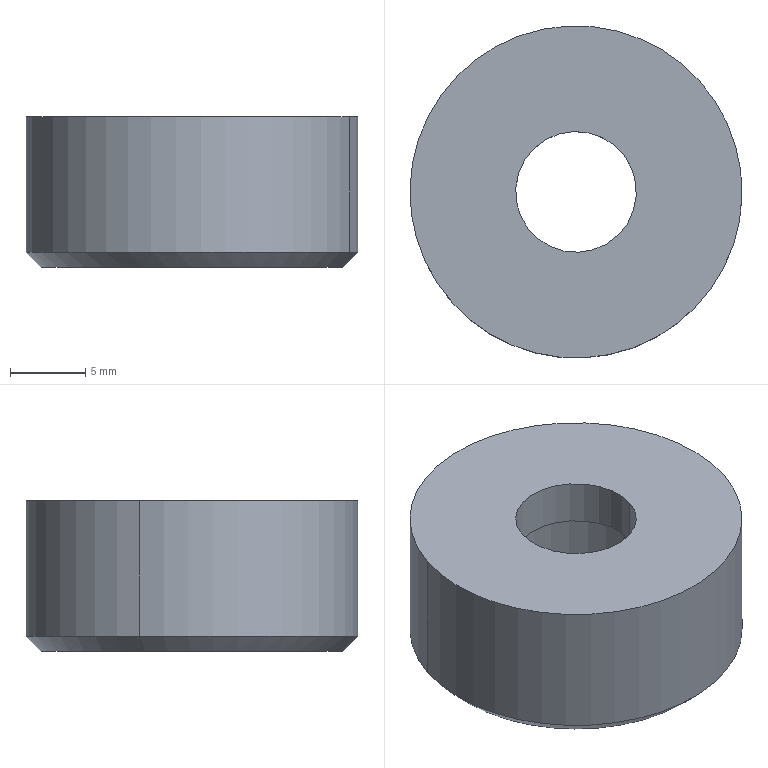Component | SolidWorks | DEM_R TEKER-1 | 1 solid | 11 faces | box 22 x 22 x 10 mm | volume 2758 mm3 | cylinder 6 | plane 3 | cone 2 | commonest cylinder face diameters 12.5 x2 22 x2 8 x2
build123d program:
from build123d import *

# Parameters (mm, degrees)
IZIM1_R                     = 11
Y_KSEKLIK_EKSTR_ZYON1_DEPTH = 10
IZIM2_R                     = 4
KES_EKSTR_ZYON1_DEPTH       = 10
IZIM3_R                     = 6.25
KES_EKSTR_ZYON2_DEPTH       = 7
CHAMFER1_SIZE               = 1


with BuildPart() as part:
    # izim1 → Y_kseklik-Ekstr_zyon1 (new body)
    with BuildSketch(Plane.XY):
        Circle(IZIM1_R)
    extrude(amount=Y_KSEKLIK_EKSTR_ZYON1_DEPTH)

    # izim2 → Kes-Ekstr_zyon1 (cut)
    with BuildSketch(Plane.XY.offset(10)):
        Circle(IZIM2_R)
    extrude(amount=-KES_EKSTR_ZYON1_DEPTH, mode=Mode.SUBTRACT)

    # izim3 → Kes-Ekstr_zyon2 (cut)
    with BuildSketch(Plane.XY.offset(10)):
        Circle(IZIM3_R)
    extrude(amount=-KES_EKSTR_ZYON2_DEPTH, mode=Mode.SUBTRACT)

    # Chamfer1
    chamfer1_edges = [part.edges().sort_by_distance(p)[0] for p in [
        (-11, 0, 10),
    ]]
    chamfer(chamfer1_edges, length=CHAMFER1_SIZE)


solid = part.part

# Placed as in the assembly
solid = solid.moved(Location((-146.473, 169.805, 183.974), (180, 0, 0)))
STEP:
#1=CARTESIAN_POINT('',(-5.393,6.561,6.849));
#2=VERTEX_POINT('',#1);
#3=CARTESIAN_POINT('',(-6.14,6.81,6.849));
#4=VERTEX_POINT('',#3);
#5=CARTESIAN_POINT('',(-5.767,6.685,6.849));
#6=DIRECTION('',(0.,-0.,-1.));
#7=DIRECTION('',(0.9488,-0.316,0.));
#8=AXIS2_PLACEMENT_3D('',#5,#6,#7);
#9=CIRCLE('',#8,0.3937);
#10=EDGE_CURVE('',#2,#4,#9,.T.);
#11=ORIENTED_EDGE('',*,*,#10,.F.);
#12=CARTESIAN_POINT('',(-5.356,6.548,6.889));
#13=VERTEX_POINT('',#12);
#14=CARTESIAN_POINT('',(-5.393,6.561,6.849));
#15=DIRECTION('',(0.6709,-0.2234,0.7071));
#16=VECTOR('',#15,39.37);
#17=LINE('',#14,#16);
#18=EDGE_CURVE('',#2,#13,#17,.T.);
#19=ORIENTED_EDGE('',*,*,#18,.T.);
#20=CARTESIAN_POINT('',(-6.178,6.822,6.889));
#21=VERTEX_POINT('',#20);
#22=CARTESIAN_POINT('',(-5.767,6.685,6.889));
#23=DIRECTION('',(-0.,0.,1.));
#24=DIRECTION('',(0.9488,-0.316,0.));
#25=AXIS2_PLACEMENT_3D('',#22,#23,#24);
#26=CIRCLE('',#25,0.4331);
#27=EDGE_CURVE('',#21,#13,#26,.T.);
#28=ORIENTED_EDGE('',*,*,#27,.F.);
#29=CARTESIAN_POINT('',(-6.14,6.81,6.849));
#30=DIRECTION('',(-0.6709,0.2234,0.7071));
#31=VECTOR('',#30,39.37);
#32=LINE('',#29,#31);
#33=EDGE_CURVE('',#4,#21,#32,.T.);
#34=ORIENTED_EDGE('',*,*,#33,.F.);
#35=EDGE_LOOP('',(#11,#19,#28,#34));
#36=FACE_OUTER_BOUND('',#35,.T.);
#37=CARTESIAN_POINT('',(-5.767,6.685,6.849));
#38=DIRECTION('',(-0.,0.,1.));
#39=DIRECTION('',(-0.9488,0.316,0.));
#40=AXIS2_PLACEMENT_3D('',#37,#38,#39);
#41=CONICAL_SURFACE('',#40,0.3937,0.7854);
#42=ADVANCED_FACE('',(#36),#41,.T.);
#43=CARTESIAN_POINT('',(-6.,6.763,7.125));
#44=VERTEX_POINT('',#43);
#45=CARTESIAN_POINT('',(-5.533,6.607,7.125));
#46=VERTEX_POINT('',#45);
#47=CARTESIAN_POINT('',(-5.767,6.685,7.125));
#48=DIRECTION('',(0.,-0.,-1.));
#49=DIRECTION('',(0.9488,-0.316,0.));
#50=AXIS2_PLACEMENT_3D('',#47,#48,#49);
#51=CIRCLE('',#50,0.2461);
#52=EDGE_CURVE('',#44,#46,#51,.T.);
#53=ORIENTED_EDGE('',*,*,#52,.F.);
#54=CARTESIAN_POINT('',(-6.,6.763,6.849));
#55=VERTEX_POINT('',#54);
#56=CARTESIAN_POINT('',(-6.,6.763,7.125));
#57=DIRECTION('',(0.,-0.,-1.));
#58=VECTOR('',#57,39.37);
#59=LINE('',#56,#58);
#60=EDGE_CURVE('',#44,#55,#59,.T.);
#61=ORIENTED_EDGE('',*,*,#60,.T.);
#62=CARTESIAN_POINT('',(-5.533,6.607,6.849));
#63=VERTEX_POINT('',#62);
#64=CARTESIAN_POINT('',(-5.767,6.685,6.849));
#65=DIRECTION('',(0.,-0.,-1.));
#66=DIRECTION('',(0.9488,-0.316,0.));
#67=AXIS2_PLACEMENT_3D('',#64,#65,#66);
#68=CIRCLE('',#67,0.2461);
#69=EDGE_CURVE('',#55,#63,#68,.T.);
#70=ORIENTED_EDGE('',*,*,#69,.T.);
#71=CARTESIAN_POINT('',(-5.533,6.607,7.125));
#72=DIRECTION('',(0.,-0.,-1.));
#73=VECTOR('',#72,39.37);
#74=LINE('',#71,#73);
#75=EDGE_CURVE('',#46,#63,#74,.T.);
#76=ORIENTED_EDGE('',*,*,#75,.F.);
#77=EDGE_LOOP('',(#53,#61,#70,#76));
#78=FACE_OUTER_BOUND('',#77,.T.);
#79=CARTESIAN_POINT('',(-5.767,6.685,7.125));
#80=DIRECTION('',(0.,-0.,-1.));
#81=DIRECTION('',(0.9488,-0.316,0.));
#82=AXIS2_PLACEMENT_3D('',#79,#80,#81);
#83=CYLINDRICAL_SURFACE('',#82,0.2461);
#84=ADVANCED_FACE('',(#78),#83,.F.);
#85=ORIENTED_EDGE('',*,*,#27,.T.);
#86=CARTESIAN_POINT('',(-5.356,6.548,7.243));
#87=VERTEX_POINT('',#86);
#88=CARTESIAN_POINT('',(-5.356,6.548,6.849));
#89=DIRECTION('',(-0.,0.,1.));
#90=VECTOR('',#89,39.37);
#91=LINE('',#88,#90);
#92=EDGE_CURVE('',#13,#87,#91,.T.);
#93=ORIENTED_EDGE('',*,*,#92,.T.);
#94=CARTESIAN_POINT('',(-6.178,6.822,7.243));
#95=VERTEX_POINT('',#94);
#96=CARTESIAN_POINT('',(-5.767,6.685,7.243));
#97=DIRECTION('',(0.,-0.,-1.));
#98=DIRECTION('',(0.9488,-0.316,0.));
#99=AXIS2_PLACEMENT_3D('',#96,#97,#98);
#100=CIRCLE('',#99,0.4331);
#101=EDGE_CURVE('',#87,#95,#100,.T.);
#102=ORIENTED_EDGE('',*,*,#101,.T.);
#103=CARTESIAN_POINT('',(-6.178,6.822,6.849));
#104=DIRECTION('',(-0.,0.,1.));
#105=VECTOR('',#104,39.37);
#106=LINE('',#103,#105);
#107=EDGE_CURVE('',#21,#95,#106,.T.);
#108=ORIENTED_EDGE('',*,*,#107,.F.);
#109=EDGE_LOOP('',(#85,#93,#102,#108));
#110=FACE_OUTER_BOUND('',#109,.T.);
#111=CARTESIAN_POINT('',(-5.767,6.685,6.849));
#112=DIRECTION('',(-0.,0.,1.));
#113=DIRECTION('',(-0.9488,0.316,0.));
#114=AXIS2_PLACEMENT_3D('',#111,#112,#113);
#115=CYLINDRICAL_SURFACE('',#114,0.4331);
#116=ADVANCED_FACE('',(#110),#115,.T.);
#117=CARTESIAN_POINT('',(-5.916,6.735,7.243));
#118=VERTEX_POINT('',#117);
#119=CARTESIAN_POINT('',(-5.617,6.635,7.243));
#120=VERTEX_POINT('',#119);
#121=CARTESIAN_POINT('',(-5.767,6.685,7.243));
#122=DIRECTION('',(0.,-0.,-1.));
#123=DIRECTION('',(0.9488,-0.316,0.));
#124=AXIS2_PLACEMENT_3D('',#121,#122,#123);
#125=CIRCLE('',#124,0.1575);
#126=EDGE_CURVE('',#118,#120,#125,.T.);
#127=ORIENTED_EDGE('',*,*,#126,.F.);
#128=CARTESIAN_POINT('',(-5.916,6.735,7.125));
#129=VERTEX_POINT('',#128);
#130=CARTESIAN_POINT('',(-5.916,6.735,7.243));
#131=DIRECTION('',(0.,-0.,-1.));
#132=VECTOR('',#131,39.37);
#133=LINE('',#130,#132);
#134=EDGE_CURVE('',#118,#129,#133,.T.);
#135=ORIENTED_EDGE('',*,*,#134,.T.);
#136=CARTESIAN_POINT('',(-5.617,6.635,7.125));
#137=VERTEX_POINT('',#136);
#138=CARTESIAN_POINT('',(-5.767,6.685,7.125));
#139=DIRECTION('',(-0.,0.,1.));
#140=DIRECTION('',(0.9488,-0.316,0.));
#141=AXIS2_PLACEMENT_3D('',#138,#139,#140);
#142=CIRCLE('',#141,0.1575);
#143=EDGE_CURVE('',#137,#129,#142,.T.);
#144=ORIENTED_EDGE('',*,*,#143,.F.);
#145=CARTESIAN_POINT('',(-5.617,6.635,7.243));
#146=DIRECTION('',(0.,-0.,-1.));
#147=VECTOR('',#146,39.37);
#148=LINE('',#145,#147);
#149=EDGE_CURVE('',#120,#137,#148,.T.);
#150=ORIENTED_EDGE('',*,*,#149,.F.);
#151=EDGE_LOOP('',(#127,#135,#144,#150));
#152=FACE_OUTER_BOUND('',#151,.T.);
#153=CARTESIAN_POINT('',(-5.767,6.685,7.243));
#154=DIRECTION('',(0.,-0.,-1.));
#155=DIRECTION('',(0.9488,-0.316,0.));
#156=AXIS2_PLACEMENT_3D('',#153,#154,#155);
#157=CYLINDRICAL_SURFACE('',#156,0.1575);
#158=ADVANCED_FACE('',(#152),#157,.F.);
#159=ORIENTED_EDGE('',*,*,#134,.F.);
#160=CARTESIAN_POINT('',(-5.767,6.685,7.243));
#161=DIRECTION('',(0.,-0.,-1.));
#162=DIRECTION('',(0.9488,-0.316,0.));
#163=AXIS2_PLACEMENT_3D('',#160,#161,#162);
#164=CIRCLE('',#163,0.1575);
#165=EDGE_CURVE('',#120,#118,#164,.T.);
#166=ORIENTED_EDGE('',*,*,#165,.F.);
#167=ORIENTED_EDGE('',*,*,#149,.T.);
#168=CARTESIAN_POINT('',(-5.767,6.685,7.125));
#169=DIRECTION('',(-0.,0.,1.));
#170=DIRECTION('',(0.9488,-0.316,0.));
#171=AXIS2_PLACEMENT_3D('',#168,#169,#170);
#172=CIRCLE('',#171,0.1575);
#173=EDGE_CURVE('',#129,#137,#172,.T.);
#174=ORIENTED_EDGE('',*,*,#173,.F.);
#175=EDGE_LOOP('',(#159,#166,#167,#174));
#176=FACE_OUTER_BOUND('',#175,.T.);
#177=CARTESIAN_POINT('',(-5.767,6.685,7.243));
#178=DIRECTION('',(0.,-0.,-1.));
#179=DIRECTION('',(0.9488,-0.316,0.));
#180=AXIS2_PLACEMENT_3D('',#177,#178,#179);
#181=CYLINDRICAL_SURFACE('',#180,0.1575);
#182=ADVANCED_FACE('',(#176),#181,.F.);
#183=ORIENTED_EDGE('',*,*,#92,.F.);
#184=CARTESIAN_POINT('',(-5.767,6.685,6.889));
#185=DIRECTION('',(-0.,0.,1.));
#186=DIRECTION('',(0.9488,-0.316,0.));
#187=AXIS2_PLACEMENT_3D('',#184,#185,#186);
#188=CIRCLE('',#187,0.4331);
#189=EDGE_CURVE('',#13,#21,#188,.T.);
#190=ORIENTED_EDGE('',*,*,#189,.T.);
#191=ORIENTED_EDGE('',*,*,#107,.T.);
#192=CARTESIAN_POINT('',(-5.767,6.685,7.243));
#193=DIRECTION('',(0.,-0.,-1.));
#194=DIRECTION('',(0.9488,-0.316,0.));
#195=AXIS2_PLACEMENT_3D('',#192,#193,#194);
#196=CIRCLE('',#195,0.4331);
#197=EDGE_CURVE('',#95,#87,#196,.T.);
#198=ORIENTED_EDGE('',*,*,#197,.T.);
#199=EDGE_LOOP('',(#183,#190,#191,#198));
#200=FACE_OUTER_BOUND('',#199,.T.);
#201=CARTESIAN_POINT('',(-5.767,6.685,6.849));
#202=DIRECTION('',(-0.,0.,1.));
#203=DIRECTION('',(-0.9488,0.316,0.));
#204=AXIS2_PLACEMENT_3D('',#201,#202,#203);
#205=CYLINDRICAL_SURFACE('',#204,0.4331);
#206=ADVANCED_FACE('',(#200),#205,.T.);
#207=CARTESIAN_POINT('',(-5.767,6.685,6.849));
#208=DIRECTION('',(0.,-0.,-1.));
#209=DIRECTION('',(0.9488,-0.316,0.));
#210=AXIS2_PLACEMENT_3D('',#207,#208,#209);
#211=CIRCLE('',#210,0.3937);
#212=EDGE_CURVE('',#4,#2,#211,.T.);
#213=ORIENTED_EDGE('',*,*,#212,.T.);
#214=ORIENTED_EDGE('',*,*,#10,.T.);
#215=EDGE_LOOP('',(#213,#214));
#216=FACE_OUTER_BOUND('',#215,.T.);
#217=CARTESIAN_POINT('',(-5.767,6.685,6.849));
#218=DIRECTION('',(0.,-0.,-1.));
#219=DIRECTION('',(0.9488,-0.316,0.));
#220=AXIS2_PLACEMENT_3D('',#217,#218,#219);
#221=CIRCLE('',#220,0.2461);
#222=EDGE_CURVE('',#63,#55,#221,.T.);
#223=ORIENTED_EDGE('',*,*,#222,.F.);
#224=ORIENTED_EDGE('',*,*,#69,.F.);
#225=EDGE_LOOP('',(#223,#224));
#226=FACE_BOUND('',#225,.T.);
#227=CARTESIAN_POINT('',(-5.767,6.685,6.849));
#228=DIRECTION('',(0.,-0.,-1.));
#229=DIRECTION('',(0.9488,-0.316,0.));
#230=AXIS2_PLACEMENT_3D('',#227,#228,#229);
#231=PLANE('',#230);
#232=ADVANCED_FACE('',(#216,#226),#231,.T.);
#233=ORIENTED_EDGE('',*,*,#165,.T.);
#234=ORIENTED_EDGE('',*,*,#126,.T.);
#235=EDGE_LOOP('',(#233,#234));
#236=FACE_BOUND('',#235,.T.);
#237=ORIENTED_EDGE('',*,*,#197,.F.);
#238=ORIENTED_EDGE('',*,*,#101,.F.);
#239=EDGE_LOOP('',(#237,#238));
#240=FACE_OUTER_BOUND('',#239,.T.);
#241=CARTESIAN_POINT('',(-5.767,6.685,7.243));
#242=DIRECTION('',(0.,-0.,-1.));
#243=DIRECTION('',(0.9488,-0.316,0.));
#244=AXIS2_PLACEMENT_3D('',#241,#242,#243);
#245=PLANE('',#244);
#246=ADVANCED_FACE('',(#236,#240),#245,.F.);
#247=CARTESIAN_POINT('',(-5.767,6.685,7.125));
#248=DIRECTION('',(0.,-0.,-1.));
#249=DIRECTION('',(0.9488,-0.316,0.));
#250=AXIS2_PLACEMENT_3D('',#247,#248,#249);
#251=CIRCLE('',#250,0.2461);
#252=EDGE_CURVE('',#46,#44,#251,.T.);
#253=ORIENTED_EDGE('',*,*,#252,.T.);
#254=ORIENTED_EDGE('',*,*,#52,.T.);
#255=EDGE_LOOP('',(#253,#254));
#256=FACE_OUTER_BOUND('',#255,.T.);
#257=ORIENTED_EDGE('',*,*,#143,.T.);
#258=ORIENTED_EDGE('',*,*,#173,.T.);
#259=EDGE_LOOP('',(#257,#258));
#260=FACE_BOUND('',#259,.T.);
#261=CARTESIAN_POINT('',(-5.767,6.685,7.125));
#262=DIRECTION('',(0.,-0.,-1.));
#263=DIRECTION('',(0.9488,-0.316,0.));
#264=AXIS2_PLACEMENT_3D('',#261,#262,#263);
#265=PLANE('',#264);
#266=ADVANCED_FACE('',(#256,#260),#265,.T.);
#267=ORIENTED_EDGE('',*,*,#60,.F.);
#268=ORIENTED_EDGE('',*,*,#252,.F.);
#269=ORIENTED_EDGE('',*,*,#75,.T.);
#270=ORIENTED_EDGE('',*,*,#222,.T.);
#271=EDGE_LOOP('',(#267,#268,#269,#270));
#272=FACE_OUTER_BOUND('',#271,.T.);
#273=CARTESIAN_POINT('',(-5.767,6.685,7.125));
#274=DIRECTION('',(0.,-0.,-1.));
#275=DIRECTION('',(0.9488,-0.316,0.));
#276=AXIS2_PLACEMENT_3D('',#273,#274,#275);
#277=CYLINDRICAL_SURFACE('',#276,0.2461);
#278=ADVANCED_FACE('',(#272),#277,.F.);
#279=ORIENTED_EDGE('',*,*,#18,.F.);
#280=ORIENTED_EDGE('',*,*,#212,.F.);
#281=ORIENTED_EDGE('',*,*,#33,.T.);
#282=ORIENTED_EDGE('',*,*,#189,.F.);
#283=EDGE_LOOP('',(#279,#280,#281,#282));
#284=FACE_OUTER_BOUND('',#283,.T.);
#285=CARTESIAN_POINT('',(-5.767,6.685,6.849));
#286=DIRECTION('',(-0.,0.,1.));
#287=DIRECTION('',(-0.9488,0.316,0.));
#288=AXIS2_PLACEMENT_3D('',#285,#286,#287);
#289=CONICAL_SURFACE('',#288,0.3937,0.7854);
#290=ADVANCED_FACE('',(#284),#289,.T.);
#291=CLOSED_SHELL('',(#42,#84,#116,#158,#182,#206,#232,#246,#266,#278,#290));
#292=MANIFOLD_SOLID_BREP('',#291);
#293=CARTESIAN_POINT('',(0.,0.,0.));
#294=DIRECTION('',(0.,0.,1.));
#295=DIRECTION('',(1.,0.,0.));
#296=AXIS2_PLACEMENT_3D('',#293,#294,#295);
#297=(LENGTH_UNIT()NAMED_UNIT(*)SI_UNIT($,.METRE.));
#298=LENGTH_MEASURE_WITH_UNIT(LENGTH_MEASURE(0.0254),#297);
#299=DIMENSIONAL_EXPONENTS(1.,0.,0.,0.,0.,0.,0.);
#300=(CONVERSION_BASED_UNIT('',#298)LENGTH_UNIT()NAMED_UNIT(#299));
#301=UNCERTAINTY_MEASURE_WITH_UNIT(LENGTH_MEASURE(0.00001),#300,'','');
#302=(NAMED_UNIT(*)PLANE_ANGLE_UNIT()SI_UNIT($,.RADIAN.));
#303=(NAMED_UNIT(*)SI_UNIT($,.STERADIAN.)SOLID_ANGLE_UNIT());
#304=(GEOMETRIC_REPRESENTATION_CONTEXT(3)GLOBAL_UNCERTAINTY_ASSIGNED_CONTEXT((#301))GLOBAL_UNIT_ASSIGNED_CONTEXT((#300,#302,#303))REPRESENTATION_CONTEXT('',''));
#305=ADVANCED_BREP_SHAPE_REPRESENTATION('',(#292,#296),#304);
#306=COLOUR_RGB('',0.7922,0.8196,0.9333);
#307=FILL_AREA_STYLE_COLOUR('',#306);
#308=FILL_AREA_STYLE('',(#307));
#309=SURFACE_STYLE_FILL_AREA(#308);
#310=SURFACE_SIDE_STYLE('',(#309));
#311=SURFACE_STYLE_USAGE(.BOTH.,#310);
#312=PRESENTATION_STYLE_ASSIGNMENT((#311));
#313=STYLED_ITEM('',(#312),#292);
#314=PRESENTATION_LAYER_ASSIGNMENT('','',(#313));
#315=(LENGTH_UNIT()NAMED_UNIT(*)SI_UNIT($,.METRE.));
#316=LENGTH_MEASURE_WITH_UNIT(LENGTH_MEASURE(0.0254),#315);
#317=DIMENSIONAL_EXPONENTS(1.,0.,0.,0.,0.,0.,0.);
#318=(CONVERSION_BASED_UNIT('',#316)LENGTH_UNIT()NAMED_UNIT(#317));
#319=UNCERTAINTY_MEASURE_WITH_UNIT(LENGTH_MEASURE(0.00001),#318,'','');
#320=(NAMED_UNIT(*)PLANE_ANGLE_UNIT()SI_UNIT($,.RADIAN.));
#321=(NAMED_UNIT(*)SI_UNIT($,.STERADIAN.)SOLID_ANGLE_UNIT());
#322=(GEOMETRIC_REPRESENTATION_CONTEXT(3)GLOBAL_UNCERTAINTY_ASSIGNED_CONTEXT((#319))GLOBAL_UNIT_ASSIGNED_CONTEXT((#318,#320,#321))REPRESENTATION_CONTEXT('',''));
#323=MECHANICAL_DESIGN_GEOMETRIC_PRESENTATION_REPRESENTATION('',(#313),#322);